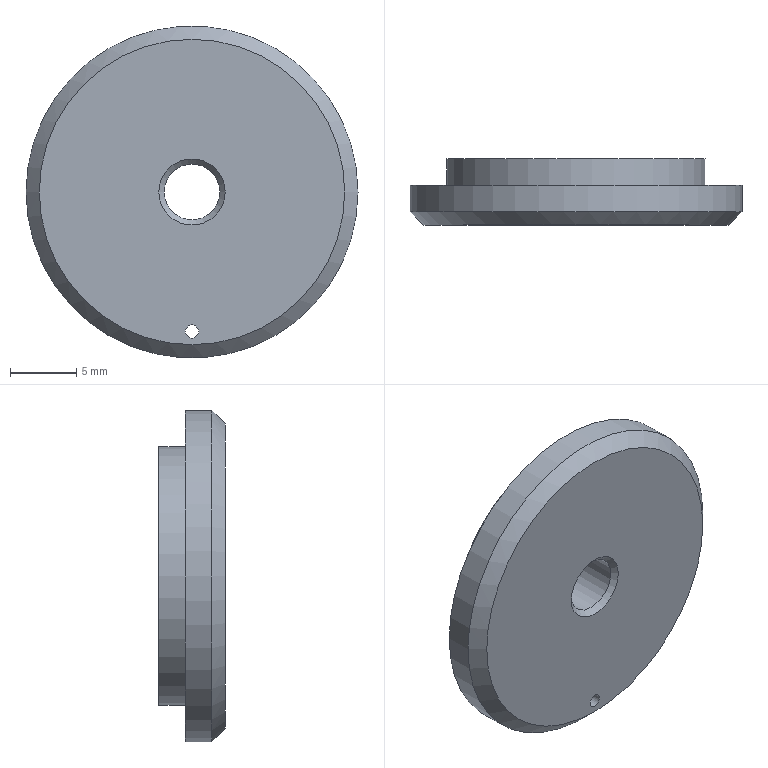Component | NX | 131_SHAFT_END_RING | 1 solid | 10 faces | box 25 x 5 x 25 mm | volume 1958 mm3 | cylinder 4 | plane 3 | cone 3 | commonest cylinder face diameters 19.5 x1 25 x1 1 x1 4.2 x1
STEP:
#1=CARTESIAN_POINT('',(0.,0.,0.));
#2=DIRECTION('',(0.,0.,1.));
#3=DIRECTION('',(1.,0.,0.));
#4=AXIS2_PLACEMENT_3D('',#1,#2,#3);
#5=CARTESIAN_POINT('',(-609.75,-183.7,-0.));
#6=VERTEX_POINT('',#5);
#7=CARTESIAN_POINT('',(-600.,-183.7,-0.));
#8=DIRECTION('',(0.,1.,0.));
#9=DIRECTION('',(-1.,0.,0.));
#10=AXIS2_PLACEMENT_3D('',#7,#8,#9);
#11=CIRCLE('',#10,9.75);
#12=CARTESIAN_POINT('',(-600.,-181.7,-0.));
#13=DIRECTION('',(0.,-1.,0.));
#14=DIRECTION('',(1.,0.,-0.));
#15=AXIS2_PLACEMENT_3D('',#12,#13,#14);
#16=CYLINDRICAL_SURFACE('',#15,9.75);
#17=CARTESIAN_POINT('',(9.425,2.));
#18=DIRECTION('',(-1.,0.));
#19=VECTOR('',#18,1.);
#20=LINE('',#17,#19);
#21=(GEOMETRIC_REPRESENTATION_CONTEXT(2)PARAMETRIC_REPRESENTATION_CONTEXT()REPRESENTATION_CONTEXT('',''));
#22=DEFINITIONAL_REPRESENTATION('',(#20),#21);
#23=PCURVE('',#16,#22);
#24=CARTESIAN_POINT('',(-600.,-183.7,-0.));
#25=DIRECTION('',(0.,1.,0.));
#26=DIRECTION('',(-1.,0.,0.));
#27=AXIS2_PLACEMENT_3D('',#24,#25,#26);
#28=PLANE('',#27);
#29=CARTESIAN_POINT('',(0.,0.));
#30=DIRECTION('',(1.,0.));
#31=AXIS2_PLACEMENT_2D('',#29,#30);
#32=CIRCLE('',#31,9.75);
#33=(GEOMETRIC_REPRESENTATION_CONTEXT(2)PARAMETRIC_REPRESENTATION_CONTEXT()REPRESENTATION_CONTEXT('',''));
#34=DEFINITIONAL_REPRESENTATION('',(#32),#33);
#35=PCURVE('',#28,#34);
#36=SURFACE_CURVE('',#11,(#23,#35),.PCURVE_S1.);
#37=EDGE_CURVE('',#6,#6,#36,.T.);
#38=ORIENTED_EDGE('',*,*,#37,.T.);
#39=CARTESIAN_POINT('',(-609.75,-181.7,-0.));
#40=VERTEX_POINT('',#39);
#41=CARTESIAN_POINT('',(-609.75,-181.7,-0.));
#42=CARTESIAN_POINT('',(-609.75,-183.7,-0.));
#43=B_SPLINE_CURVE_WITH_KNOTS('',1,(#41,#42),.UNSPECIFIED.,.F.,.F.,(2,2),(0.,2.),.PIECEWISE_BEZIER_KNOTS.);
#44=CARTESIAN_POINT('',(3.142,0.));
#45=DIRECTION('',(0.,1.));
#46=VECTOR('',#45,1.);
#47=LINE('',#44,#46);
#48=(GEOMETRIC_REPRESENTATION_CONTEXT(2)PARAMETRIC_REPRESENTATION_CONTEXT()REPRESENTATION_CONTEXT('',''));
#49=DEFINITIONAL_REPRESENTATION('',(#47),#48);
#50=PCURVE('',#16,#49);
#51=CARTESIAN_POINT('',(9.425,0.));
#52=DIRECTION('',(0.,1.));
#53=VECTOR('',#52,1.);
#54=LINE('',#51,#53);
#55=(GEOMETRIC_REPRESENTATION_CONTEXT(2)PARAMETRIC_REPRESENTATION_CONTEXT()REPRESENTATION_CONTEXT('',''));
#56=DEFINITIONAL_REPRESENTATION('',(#54),#55);
#57=PCURVE('',#16,#56);
#58=SEAM_CURVE('',#43,(#50,#57),.PCURVE_S1.);
#59=EDGE_CURVE('',#40,#6,#58,.T.);
#60=ORIENTED_EDGE('',*,*,#59,.F.);
#61=CARTESIAN_POINT('',(-600.,-181.7,-0.));
#62=DIRECTION('',(0.,1.,0.));
#63=DIRECTION('',(-1.,0.,0.));
#64=AXIS2_PLACEMENT_3D('',#61,#62,#63);
#65=CIRCLE('',#64,9.75);
#66=CARTESIAN_POINT('',(9.425,0.));
#67=DIRECTION('',(-1.,0.));
#68=VECTOR('',#67,1.);
#69=LINE('',#66,#68);
#70=(GEOMETRIC_REPRESENTATION_CONTEXT(2)PARAMETRIC_REPRESENTATION_CONTEXT()REPRESENTATION_CONTEXT('',''));
#71=DEFINITIONAL_REPRESENTATION('',(#69),#70);
#72=PCURVE('',#16,#71);
#73=CARTESIAN_POINT('',(-600.,-181.7,-0.));
#74=DIRECTION('',(0.,1.,0.));
#75=DIRECTION('',(-1.,0.,0.));
#76=AXIS2_PLACEMENT_3D('',#73,#74,#75);
#77=PLANE('',#76);
#78=CARTESIAN_POINT('',(0.,0.));
#79=DIRECTION('',(1.,0.));
#80=AXIS2_PLACEMENT_2D('',#78,#79);
#81=CIRCLE('',#80,9.75);
#82=(GEOMETRIC_REPRESENTATION_CONTEXT(2)PARAMETRIC_REPRESENTATION_CONTEXT()REPRESENTATION_CONTEXT('',''));
#83=DEFINITIONAL_REPRESENTATION('',(#81),#82);
#84=PCURVE('',#77,#83);
#85=SURFACE_CURVE('',#65,(#72,#84),.PCURVE_S1.);
#86=EDGE_CURVE('',#40,#40,#85,.T.);
#87=ORIENTED_EDGE('',*,*,#86,.F.);
#88=ORIENTED_EDGE('',*,*,#59,.T.);
#89=EDGE_LOOP('',(#38,#60,#87,#88));
#90=FACE_BOUND('',#89,.T.);
#91=ADVANCED_FACE('',(#90),#16,.T.);
#92=CARTESIAN_POINT('',(-602.5,-181.7,-0.));
#93=VERTEX_POINT('',#92);
#94=CARTESIAN_POINT('',(-600.,-181.7,-0.));
#95=DIRECTION('',(0.,-1.,0.));
#96=DIRECTION('',(-1.,0.,0.));
#97=AXIS2_PLACEMENT_3D('',#94,#95,#96);
#98=CIRCLE('',#97,2.5);
#99=CARTESIAN_POINT('',(2.5,0.));
#100=CARTESIAN_POINT('',(2.5,-4.33));
#101=CARTESIAN_POINT('',(-1.25,-2.165));
#102=CARTESIAN_POINT('',(-5.,-0.));
#103=CARTESIAN_POINT('',(-1.25,2.165));
#104=CARTESIAN_POINT('',(2.5,4.33));
#105=CARTESIAN_POINT('',(2.5,0.));
#106=(BOUNDED_CURVE()B_SPLINE_CURVE(2,(#99,#100,#101,#102,#103,#104,#105),.UNSPECIFIED.,.T.,.F.)B_SPLINE_CURVE_WITH_KNOTS((1,2,2,2,2,1),(-2.094,0.,2.094,4.189,6.283,8.378),.UNSPECIFIED.)CURVE()GEOMETRIC_REPRESENTATION_ITEM()RATIONAL_B_SPLINE_CURVE((1.,0.5,1.,0.5,1.,0.5,1.))REPRESENTATION_ITEM(''));
#107=(GEOMETRIC_REPRESENTATION_CONTEXT(2)PARAMETRIC_REPRESENTATION_CONTEXT()REPRESENTATION_CONTEXT('',''));
#108=DEFINITIONAL_REPRESENTATION('',(#106),#107);
#109=PCURVE('',#77,#108);
#110=CARTESIAN_POINT('',(-600.,-182.1,-0.));
#111=DIRECTION('',(0.,1.,0.));
#112=DIRECTION('',(-1.,0.,0.));
#113=AXIS2_PLACEMENT_3D('',#110,#111,#112);
#114=CONICAL_SURFACE('',#113,2.1,0.7854);
#115=CARTESIAN_POINT('',(6.283,0.4));
#116=DIRECTION('',(-1.,0.));
#117=VECTOR('',#116,1.);
#118=LINE('',#115,#117);
#119=(GEOMETRIC_REPRESENTATION_CONTEXT(2)PARAMETRIC_REPRESENTATION_CONTEXT()REPRESENTATION_CONTEXT('',''));
#120=DEFINITIONAL_REPRESENTATION('',(#118),#119);
#121=PCURVE('',#114,#120);
#122=SURFACE_CURVE('',#98,(#109,#121),.PCURVE_S1.);
#123=EDGE_CURVE('',#93,#93,#122,.T.);
#124=ORIENTED_EDGE('',*,*,#123,.T.);
#125=EDGE_LOOP('',(#124));
#126=FACE_BOUND('',#125,.T.);
#127=ORIENTED_EDGE('',*,*,#86,.T.);
#128=EDGE_LOOP('',(#127));
#129=FACE_BOUND('',#128,.T.);
#130=ADVANCED_FACE('',(#126,#129),#77,.T.);
#131=CARTESIAN_POINT('',(-612.5,-185.7,-0.));
#132=VERTEX_POINT('',#131);
#133=CARTESIAN_POINT('',(-600.,-185.7,-0.));
#134=DIRECTION('',(0.,1.,0.));
#135=DIRECTION('',(-1.,0.,0.));
#136=AXIS2_PLACEMENT_3D('',#133,#134,#135);
#137=CIRCLE('',#136,12.5);
#138=CARTESIAN_POINT('',(-600.,-183.7,-0.));
#139=DIRECTION('',(0.,-1.,0.));
#140=DIRECTION('',(1.,0.,-0.));
#141=AXIS2_PLACEMENT_3D('',#138,#139,#140);
#142=CYLINDRICAL_SURFACE('',#141,12.5);
#143=CARTESIAN_POINT('',(9.425,2.));
#144=DIRECTION('',(-1.,0.));
#145=VECTOR('',#144,1.);
#146=LINE('',#143,#145);
#147=(GEOMETRIC_REPRESENTATION_CONTEXT(2)PARAMETRIC_REPRESENTATION_CONTEXT()REPRESENTATION_CONTEXT('',''));
#148=DEFINITIONAL_REPRESENTATION('',(#146),#147);
#149=PCURVE('',#142,#148);
#150=CARTESIAN_POINT('',(-600.,-185.7,-0.));
#151=DIRECTION('',(0.,1.,0.));
#152=DIRECTION('',(-1.,0.,0.));
#153=AXIS2_PLACEMENT_3D('',#150,#151,#152);
#154=CONICAL_SURFACE('',#153,12.5,0.7854);
#155=CARTESIAN_POINT('',(0.,0.));
#156=DIRECTION('',(1.,0.));
#157=VECTOR('',#156,1.);
#158=LINE('',#155,#157);
#159=(GEOMETRIC_REPRESENTATION_CONTEXT(2)PARAMETRIC_REPRESENTATION_CONTEXT()REPRESENTATION_CONTEXT('',''));
#160=DEFINITIONAL_REPRESENTATION('',(#158),#159);
#161=PCURVE('',#154,#160);
#162=SURFACE_CURVE('',#137,(#149,#161),.PCURVE_S1.);
#163=EDGE_CURVE('',#132,#132,#162,.T.);
#164=ORIENTED_EDGE('',*,*,#163,.T.);
#165=CARTESIAN_POINT('',(-612.5,-183.7,-0.));
#166=VERTEX_POINT('',#165);
#167=CARTESIAN_POINT('',(-612.5,-183.7,-0.));
#168=CARTESIAN_POINT('',(-612.5,-185.7,-0.));
#169=B_SPLINE_CURVE_WITH_KNOTS('',1,(#167,#168),.UNSPECIFIED.,.F.,.F.,(2,2),(0.,2.),.PIECEWISE_BEZIER_KNOTS.);
#170=CARTESIAN_POINT('',(3.142,0.));
#171=DIRECTION('',(0.,1.));
#172=VECTOR('',#171,1.);
#173=LINE('',#170,#172);
#174=(GEOMETRIC_REPRESENTATION_CONTEXT(2)PARAMETRIC_REPRESENTATION_CONTEXT()REPRESENTATION_CONTEXT('',''));
#175=DEFINITIONAL_REPRESENTATION('',(#173),#174);
#176=PCURVE('',#142,#175);
#177=CARTESIAN_POINT('',(9.425,0.));
#178=DIRECTION('',(0.,1.));
#179=VECTOR('',#178,1.);
#180=LINE('',#177,#179);
#181=(GEOMETRIC_REPRESENTATION_CONTEXT(2)PARAMETRIC_REPRESENTATION_CONTEXT()REPRESENTATION_CONTEXT('',''));
#182=DEFINITIONAL_REPRESENTATION('',(#180),#181);
#183=PCURVE('',#142,#182);
#184=SEAM_CURVE('',#169,(#176,#183),.PCURVE_S1.);
#185=EDGE_CURVE('',#166,#132,#184,.T.);
#186=ORIENTED_EDGE('',*,*,#185,.F.);
#187=CARTESIAN_POINT('',(-600.,-183.7,-0.));
#188=DIRECTION('',(0.,1.,0.));
#189=DIRECTION('',(-1.,0.,0.));
#190=AXIS2_PLACEMENT_3D('',#187,#188,#189);
#191=CIRCLE('',#190,12.5);
#192=CARTESIAN_POINT('',(9.425,0.));
#193=DIRECTION('',(-1.,0.));
#194=VECTOR('',#193,1.);
#195=LINE('',#192,#194);
#196=(GEOMETRIC_REPRESENTATION_CONTEXT(2)PARAMETRIC_REPRESENTATION_CONTEXT()REPRESENTATION_CONTEXT('',''));
#197=DEFINITIONAL_REPRESENTATION('',(#195),#196);
#198=PCURVE('',#142,#197);
#199=CARTESIAN_POINT('',(0.,0.));
#200=DIRECTION('',(1.,0.));
#201=AXIS2_PLACEMENT_2D('',#199,#200);
#202=CIRCLE('',#201,12.5);
#203=(GEOMETRIC_REPRESENTATION_CONTEXT(2)PARAMETRIC_REPRESENTATION_CONTEXT()REPRESENTATION_CONTEXT('',''));
#204=DEFINITIONAL_REPRESENTATION('',(#202),#203);
#205=PCURVE('',#28,#204);
#206=SURFACE_CURVE('',#191,(#198,#205),.PCURVE_S1.);
#207=EDGE_CURVE('',#166,#166,#206,.T.);
#208=ORIENTED_EDGE('',*,*,#207,.F.);
#209=ORIENTED_EDGE('',*,*,#185,.T.);
#210=EDGE_LOOP('',(#164,#186,#208,#209));
#211=FACE_BOUND('',#210,.T.);
#212=ADVANCED_FACE('',(#211),#142,.T.);
#213=CARTESIAN_POINT('',(-600.5,-183.7,-10.5));
#214=VERTEX_POINT('',#213);
#215=CARTESIAN_POINT('',(-600.,-183.7,-10.5));
#216=DIRECTION('',(0.,1.,0.));
#217=DIRECTION('',(-1.,0.,0.));
#218=AXIS2_PLACEMENT_3D('',#215,#216,#217);
#219=CIRCLE('',#218,0.5);
#220=CARTESIAN_POINT('',(0.,-10.5));
#221=DIRECTION('',(1.,0.));
#222=AXIS2_PLACEMENT_2D('',#220,#221);
#223=CIRCLE('',#222,0.5);
#224=(GEOMETRIC_REPRESENTATION_CONTEXT(2)PARAMETRIC_REPRESENTATION_CONTEXT()REPRESENTATION_CONTEXT('',''));
#225=DEFINITIONAL_REPRESENTATION('',(#223),#224);
#226=PCURVE('',#28,#225);
#227=CARTESIAN_POINT('',(-600.,-181.7,-10.5));
#228=DIRECTION('',(0.,-1.,0.));
#229=DIRECTION('',(1.,0.,-0.));
#230=AXIS2_PLACEMENT_3D('',#227,#228,#229);
#231=CYLINDRICAL_SURFACE('',#230,0.5);
#232=CARTESIAN_POINT('',(9.425,2.));
#233=DIRECTION('',(-1.,0.));
#234=VECTOR('',#233,1.);
#235=LINE('',#232,#234);
#236=(GEOMETRIC_REPRESENTATION_CONTEXT(2)PARAMETRIC_REPRESENTATION_CONTEXT()REPRESENTATION_CONTEXT('',''));
#237=DEFINITIONAL_REPRESENTATION('',(#235),#236);
#238=PCURVE('',#231,#237);
#239=SURFACE_CURVE('',#219,(#226,#238),.PCURVE_S1.);
#240=EDGE_CURVE('',#214,#214,#239,.T.);
#241=ORIENTED_EDGE('',*,*,#240,.F.);
#242=EDGE_LOOP('',(#241));
#243=FACE_BOUND('',#242,.T.);
#244=ORIENTED_EDGE('',*,*,#207,.T.);
#245=EDGE_LOOP('',(#244));
#246=FACE_BOUND('',#245,.T.);
#247=ORIENTED_EDGE('',*,*,#37,.F.);
#248=EDGE_LOOP('',(#247));
#249=FACE_BOUND('',#248,.T.);
#250=ADVANCED_FACE('',(#243,#246,#249),#28,.T.);
#251=CARTESIAN_POINT('',(-602.5,-186.7,-0.));
#252=VERTEX_POINT('',#251);
#253=CARTESIAN_POINT('',(-600.,-186.7,-0.));
#254=DIRECTION('',(0.,1.,0.));
#255=DIRECTION('',(-1.,0.,0.));
#256=AXIS2_PLACEMENT_3D('',#253,#254,#255);
#257=CIRCLE('',#256,2.5);
#258=CARTESIAN_POINT('',(-600.,-186.7,-0.));
#259=DIRECTION('',(0.,1.,0.));
#260=DIRECTION('',(-1.,0.,0.));
#261=AXIS2_PLACEMENT_3D('',#258,#259,#260);
#262=PLANE('',#261);
#263=CARTESIAN_POINT('',(0.,0.));
#264=DIRECTION('',(1.,0.));
#265=AXIS2_PLACEMENT_2D('',#263,#264);
#266=CIRCLE('',#265,2.5);
#267=(GEOMETRIC_REPRESENTATION_CONTEXT(2)PARAMETRIC_REPRESENTATION_CONTEXT()REPRESENTATION_CONTEXT('',''));
#268=DEFINITIONAL_REPRESENTATION('',(#266),#267);
#269=PCURVE('',#262,#268);
#270=CARTESIAN_POINT('',(-600.,-186.7,-0.));
#271=DIRECTION('',(0.,-1.,0.));
#272=DIRECTION('',(1.,0.,-0.));
#273=AXIS2_PLACEMENT_3D('',#270,#271,#272);
#274=CONICAL_SURFACE('',#273,2.5,0.7854);
#275=CARTESIAN_POINT('',(9.425,0.));
#276=DIRECTION('',(-1.,0.));
#277=VECTOR('',#276,1.);
#278=LINE('',#275,#277);
#279=(GEOMETRIC_REPRESENTATION_CONTEXT(2)PARAMETRIC_REPRESENTATION_CONTEXT()REPRESENTATION_CONTEXT('',''));
#280=DEFINITIONAL_REPRESENTATION('',(#278),#279);
#281=PCURVE('',#274,#280);
#282=SURFACE_CURVE('',#257,(#269,#281),.PCURVE_S1.);
#283=EDGE_CURVE('',#252,#252,#282,.T.);
#284=ORIENTED_EDGE('',*,*,#283,.T.);
#285=EDGE_LOOP('',(#284));
#286=FACE_BOUND('',#285,.T.);
#287=CARTESIAN_POINT('',(-600.5,-186.7,-10.5));
#288=VERTEX_POINT('',#287);
#289=CARTESIAN_POINT('',(-600.,-186.7,-10.5));
#290=DIRECTION('',(0.,-1.,0.));
#291=DIRECTION('',(-1.,0.,0.));
#292=AXIS2_PLACEMENT_3D('',#289,#290,#291);
#293=CIRCLE('',#292,0.5);
#294=CARTESIAN_POINT('',(0.5,-10.5));
#295=CARTESIAN_POINT('',(0.5,-11.366));
#296=CARTESIAN_POINT('',(-0.25,-10.933));
#297=CARTESIAN_POINT('',(-1.,-10.5));
#298=CARTESIAN_POINT('',(-0.25,-10.067));
#299=CARTESIAN_POINT('',(0.5,-9.634));
#300=CARTESIAN_POINT('',(0.5,-10.5));
#301=(BOUNDED_CURVE()B_SPLINE_CURVE(2,(#294,#295,#296,#297,#298,#299,#300),.UNSPECIFIED.,.T.,.F.)B_SPLINE_CURVE_WITH_KNOTS((1,2,2,2,2,1),(-2.094,0.,2.094,4.189,6.283,8.378),.UNSPECIFIED.)CURVE()GEOMETRIC_REPRESENTATION_ITEM()RATIONAL_B_SPLINE_CURVE((1.,0.5,1.,0.5,1.,0.5,1.))REPRESENTATION_ITEM(''));
#302=(GEOMETRIC_REPRESENTATION_CONTEXT(2)PARAMETRIC_REPRESENTATION_CONTEXT()REPRESENTATION_CONTEXT('',''));
#303=DEFINITIONAL_REPRESENTATION('',(#301),#302);
#304=PCURVE('',#262,#303);
#305=CARTESIAN_POINT('',(3.142,5.));
#306=DIRECTION('',(1.,0.));
#307=VECTOR('',#306,1.);
#308=LINE('',#305,#307);
#309=(GEOMETRIC_REPRESENTATION_CONTEXT(2)PARAMETRIC_REPRESENTATION_CONTEXT()REPRESENTATION_CONTEXT('',''));
#310=DEFINITIONAL_REPRESENTATION('',(#308),#309);
#311=PCURVE('',#231,#310);
#312=SURFACE_CURVE('',#293,(#304,#311),.PCURVE_S1.);
#313=EDGE_CURVE('',#288,#288,#312,.T.);
#314=ORIENTED_EDGE('',*,*,#313,.F.);
#315=EDGE_LOOP('',(#314));
#316=FACE_BOUND('',#315,.T.);
#317=CARTESIAN_POINT('',(-611.5,-186.7,-0.));
#318=VERTEX_POINT('',#317);
#319=CARTESIAN_POINT('',(-600.,-186.7,-0.));
#320=DIRECTION('',(0.,-1.,0.));
#321=DIRECTION('',(-1.,0.,0.));
#322=AXIS2_PLACEMENT_3D('',#319,#320,#321);
#323=CIRCLE('',#322,11.5);
#324=CARTESIAN_POINT('',(11.5,0.));
#325=CARTESIAN_POINT('',(11.5,-19.919));
#326=CARTESIAN_POINT('',(-5.75,-9.959));
#327=CARTESIAN_POINT('',(-23.,-0.));
#328=CARTESIAN_POINT('',(-5.75,9.959));
#329=CARTESIAN_POINT('',(11.5,19.919));
#330=CARTESIAN_POINT('',(11.5,0.));
#331=(BOUNDED_CURVE()B_SPLINE_CURVE(2,(#324,#325,#326,#327,#328,#329,#330),.UNSPECIFIED.,.T.,.F.)B_SPLINE_CURVE_WITH_KNOTS((1,2,2,2,2,1),(-2.094,0.,2.094,4.189,6.283,8.378),.UNSPECIFIED.)CURVE()GEOMETRIC_REPRESENTATION_ITEM()RATIONAL_B_SPLINE_CURVE((1.,0.5,1.,0.5,1.,0.5,1.))REPRESENTATION_ITEM(''));
#332=(GEOMETRIC_REPRESENTATION_CONTEXT(2)PARAMETRIC_REPRESENTATION_CONTEXT()REPRESENTATION_CONTEXT('',''));
#333=DEFINITIONAL_REPRESENTATION('',(#331),#332);
#334=PCURVE('',#262,#333);
#335=CARTESIAN_POINT('',(6.283,-1.));
#336=DIRECTION('',(-1.,0.));
#337=VECTOR('',#336,1.);
#338=LINE('',#335,#337);
#339=(GEOMETRIC_REPRESENTATION_CONTEXT(2)PARAMETRIC_REPRESENTATION_CONTEXT()REPRESENTATION_CONTEXT('',''));
#340=DEFINITIONAL_REPRESENTATION('',(#338),#339);
#341=PCURVE('',#154,#340);
#342=SURFACE_CURVE('',#323,(#334,#341),.PCURVE_S1.);
#343=EDGE_CURVE('',#318,#318,#342,.T.);
#344=ORIENTED_EDGE('',*,*,#343,.T.);
#345=EDGE_LOOP('',(#344));
#346=FACE_BOUND('',#345,.T.);
#347=ADVANCED_FACE('',(#286,#316,#346),#262,.F.);
#348=ORIENTED_EDGE('',*,*,#343,.F.);
#349=CARTESIAN_POINT('',(-611.5,-186.7,-0.));
#350=CARTESIAN_POINT('',(-612.5,-185.7,-0.));
#351=B_SPLINE_CURVE_WITH_KNOTS('',1,(#349,#350),.UNSPECIFIED.,.F.,.F.,(2,2),(-1.414,0.),.PIECEWISE_BEZIER_KNOTS.);
#352=CARTESIAN_POINT('',(6.283,0.));
#353=DIRECTION('',(0.,1.));
#354=VECTOR('',#353,1.);
#355=LINE('',#352,#354);
#356=(GEOMETRIC_REPRESENTATION_CONTEXT(2)PARAMETRIC_REPRESENTATION_CONTEXT()REPRESENTATION_CONTEXT('',''));
#357=DEFINITIONAL_REPRESENTATION('',(#355),#356);
#358=PCURVE('',#154,#357);
#359=CARTESIAN_POINT('',(0.,0.));
#360=DIRECTION('',(0.,1.));
#361=VECTOR('',#360,1.);
#362=LINE('',#359,#361);
#363=(GEOMETRIC_REPRESENTATION_CONTEXT(2)PARAMETRIC_REPRESENTATION_CONTEXT()REPRESENTATION_CONTEXT('',''));
#364=DEFINITIONAL_REPRESENTATION('',(#362),#363);
#365=PCURVE('',#154,#364);
#366=SEAM_CURVE('',#351,(#358,#365),.PCURVE_S1.);
#367=EDGE_CURVE('',#318,#132,#366,.T.);
#368=ORIENTED_EDGE('',*,*,#367,.T.);
#369=ORIENTED_EDGE('',*,*,#163,.F.);
#370=ORIENTED_EDGE('',*,*,#367,.F.);
#371=EDGE_LOOP('',(#348,#368,#369,#370));
#372=FACE_BOUND('',#371,.T.);
#373=ADVANCED_FACE('',(#372),#154,.T.);
#374=ORIENTED_EDGE('',*,*,#240,.F.);
#375=CARTESIAN_POINT('',(-600.5,-183.7,-10.5));
#376=CARTESIAN_POINT('',(-600.5,-186.7,-10.5));
#377=B_SPLINE_CURVE_WITH_KNOTS('',1,(#375,#376),.UNSPECIFIED.,.F.,.F.,(2,2),(2.,5.),.PIECEWISE_BEZIER_KNOTS.);
#378=CARTESIAN_POINT('',(9.425,0.));
#379=DIRECTION('',(0.,1.));
#380=VECTOR('',#379,1.);
#381=LINE('',#378,#380);
#382=(GEOMETRIC_REPRESENTATION_CONTEXT(2)PARAMETRIC_REPRESENTATION_CONTEXT()REPRESENTATION_CONTEXT('',''));
#383=DEFINITIONAL_REPRESENTATION('',(#381),#382);
#384=PCURVE('',#231,#383);
#385=CARTESIAN_POINT('',(3.142,0.));
#386=DIRECTION('',(0.,1.));
#387=VECTOR('',#386,1.);
#388=LINE('',#385,#387);
#389=(GEOMETRIC_REPRESENTATION_CONTEXT(2)PARAMETRIC_REPRESENTATION_CONTEXT()REPRESENTATION_CONTEXT('',''));
#390=DEFINITIONAL_REPRESENTATION('',(#388),#389);
#391=PCURVE('',#231,#390);
#392=SEAM_CURVE('',#377,(#384,#391),.PCURVE_S1.);
#393=EDGE_CURVE('',#214,#288,#392,.T.);
#394=ORIENTED_EDGE('',*,*,#393,.T.);
#395=ORIENTED_EDGE('',*,*,#313,.F.);
#396=ORIENTED_EDGE('',*,*,#393,.F.);
#397=EDGE_LOOP('',(#374,#394,#395,#396));
#398=FACE_BOUND('',#397,.F.);
#399=ADVANCED_FACE('',(#398),#231,.F.);
#400=CARTESIAN_POINT('',(-602.1,-182.1,-0.));
#401=VERTEX_POINT('',#400);
#402=CARTESIAN_POINT('',(-600.,-182.1,-0.));
#403=DIRECTION('',(0.,1.,0.));
#404=DIRECTION('',(-1.,0.,0.));
#405=AXIS2_PLACEMENT_3D('',#402,#403,#404);
#406=CIRCLE('',#405,2.1);
#407=CARTESIAN_POINT('',(-600.,-186.7,-0.));
#408=DIRECTION('',(0.,1.,0.));
#409=DIRECTION('',(-1.,0.,0.));
#410=AXIS2_PLACEMENT_3D('',#407,#408,#409);
#411=CYLINDRICAL_SURFACE('',#410,2.1);
#412=CARTESIAN_POINT('',(0.,4.6));
#413=DIRECTION('',(1.,0.));
#414=VECTOR('',#413,1.);
#415=LINE('',#412,#414);
#416=(GEOMETRIC_REPRESENTATION_CONTEXT(2)PARAMETRIC_REPRESENTATION_CONTEXT()REPRESENTATION_CONTEXT('',''));
#417=DEFINITIONAL_REPRESENTATION('',(#415),#416);
#418=PCURVE('',#411,#417);
#419=CARTESIAN_POINT('',(0.,0.));
#420=DIRECTION('',(1.,0.));
#421=VECTOR('',#420,1.);
#422=LINE('',#419,#421);
#423=(GEOMETRIC_REPRESENTATION_CONTEXT(2)PARAMETRIC_REPRESENTATION_CONTEXT()REPRESENTATION_CONTEXT('',''));
#424=DEFINITIONAL_REPRESENTATION('',(#422),#423);
#425=PCURVE('',#114,#424);
#426=SURFACE_CURVE('',#406,(#418,#425),.PCURVE_S1.);
#427=EDGE_CURVE('',#401,#401,#426,.T.);
#428=ORIENTED_EDGE('',*,*,#427,.F.);
#429=CARTESIAN_POINT('',(-602.1,-186.3,-0.));
#430=VERTEX_POINT('',#429);
#431=CARTESIAN_POINT('',(-602.1,-186.3,-0.));
#432=CARTESIAN_POINT('',(-602.1,-182.1,-0.));
#433=B_SPLINE_CURVE_WITH_KNOTS('',1,(#431,#432),.UNSPECIFIED.,.F.,.F.,(2,2),(0.4,4.6),.PIECEWISE_BEZIER_KNOTS.);
#434=CARTESIAN_POINT('',(0.,0.));
#435=DIRECTION('',(0.,1.));
#436=VECTOR('',#435,1.);
#437=LINE('',#434,#436);
#438=(GEOMETRIC_REPRESENTATION_CONTEXT(2)PARAMETRIC_REPRESENTATION_CONTEXT()REPRESENTATION_CONTEXT('',''));
#439=DEFINITIONAL_REPRESENTATION('',(#437),#438);
#440=PCURVE('',#411,#439);
#441=CARTESIAN_POINT('',(6.283,0.));
#442=DIRECTION('',(0.,1.));
#443=VECTOR('',#442,1.);
#444=LINE('',#441,#443);
#445=(GEOMETRIC_REPRESENTATION_CONTEXT(2)PARAMETRIC_REPRESENTATION_CONTEXT()REPRESENTATION_CONTEXT('',''));
#446=DEFINITIONAL_REPRESENTATION('',(#444),#445);
#447=PCURVE('',#411,#446);
#448=SEAM_CURVE('',#433,(#440,#447),.PCURVE_S1.);
#449=EDGE_CURVE('',#430,#401,#448,.T.);
#450=ORIENTED_EDGE('',*,*,#449,.F.);
#451=CARTESIAN_POINT('',(-600.,-186.3,-0.));
#452=DIRECTION('',(0.,-1.,0.));
#453=DIRECTION('',(-1.,0.,0.));
#454=AXIS2_PLACEMENT_3D('',#451,#452,#453);
#455=CIRCLE('',#454,2.1);
#456=CARTESIAN_POINT('',(6.283,0.4));
#457=DIRECTION('',(-1.,0.));
#458=VECTOR('',#457,1.);
#459=LINE('',#456,#458);
#460=(GEOMETRIC_REPRESENTATION_CONTEXT(2)PARAMETRIC_REPRESENTATION_CONTEXT()REPRESENTATION_CONTEXT('',''));
#461=DEFINITIONAL_REPRESENTATION('',(#459),#460);
#462=PCURVE('',#411,#461);
#463=CARTESIAN_POINT('',(3.142,-0.4));
#464=DIRECTION('',(1.,0.));
#465=VECTOR('',#464,1.);
#466=LINE('',#463,#465);
#467=(GEOMETRIC_REPRESENTATION_CONTEXT(2)PARAMETRIC_REPRESENTATION_CONTEXT()REPRESENTATION_CONTEXT('',''));
#468=DEFINITIONAL_REPRESENTATION('',(#466),#467);
#469=PCURVE('',#274,#468);
#470=SURFACE_CURVE('',#455,(#462,#469),.PCURVE_S1.);
#471=EDGE_CURVE('',#430,#430,#470,.T.);
#472=ORIENTED_EDGE('',*,*,#471,.F.);
#473=ORIENTED_EDGE('',*,*,#449,.T.);
#474=EDGE_LOOP('',(#428,#450,#472,#473));
#475=FACE_BOUND('',#474,.F.);
#476=ADVANCED_FACE('',(#475),#411,.F.);
#477=ORIENTED_EDGE('',*,*,#471,.T.);
#478=CARTESIAN_POINT('',(-602.1,-186.3,-0.));
#479=CARTESIAN_POINT('',(-602.5,-186.7,-0.));
#480=B_SPLINE_CURVE_WITH_KNOTS('',1,(#478,#479),.UNSPECIFIED.,.F.,.F.,(2,2),(-0.5657,0.),.PIECEWISE_BEZIER_KNOTS.);
#481=CARTESIAN_POINT('',(9.425,0.));
#482=DIRECTION('',(0.,1.));
#483=VECTOR('',#482,1.);
#484=LINE('',#481,#483);
#485=(GEOMETRIC_REPRESENTATION_CONTEXT(2)PARAMETRIC_REPRESENTATION_CONTEXT()REPRESENTATION_CONTEXT('',''));
#486=DEFINITIONAL_REPRESENTATION('',(#484),#485);
#487=PCURVE('',#274,#486);
#488=CARTESIAN_POINT('',(3.142,0.));
#489=DIRECTION('',(0.,1.));
#490=VECTOR('',#489,1.);
#491=LINE('',#488,#490);
#492=(GEOMETRIC_REPRESENTATION_CONTEXT(2)PARAMETRIC_REPRESENTATION_CONTEXT()REPRESENTATION_CONTEXT('',''));
#493=DEFINITIONAL_REPRESENTATION('',(#491),#492);
#494=PCURVE('',#274,#493);
#495=SEAM_CURVE('',#480,(#487,#494),.PCURVE_S1.);
#496=EDGE_CURVE('',#430,#252,#495,.T.);
#497=ORIENTED_EDGE('',*,*,#496,.T.);
#498=ORIENTED_EDGE('',*,*,#283,.T.);
#499=ORIENTED_EDGE('',*,*,#496,.F.);
#500=EDGE_LOOP('',(#477,#497,#498,#499));
#501=FACE_BOUND('',#500,.F.);
#502=ADVANCED_FACE('',(#501),#274,.F.);
#503=ORIENTED_EDGE('',*,*,#123,.T.);
#504=CARTESIAN_POINT('',(-602.1,-182.1,-0.));
#505=CARTESIAN_POINT('',(-602.5,-181.7,-0.));
#506=B_SPLINE_CURVE_WITH_KNOTS('',1,(#504,#505),.UNSPECIFIED.,.F.,.F.,(2,2),(0.,0.5657),.PIECEWISE_BEZIER_KNOTS.);
#507=CARTESIAN_POINT('',(0.,0.));
#508=DIRECTION('',(0.,1.));
#509=VECTOR('',#508,1.);
#510=LINE('',#507,#509);
#511=(GEOMETRIC_REPRESENTATION_CONTEXT(2)PARAMETRIC_REPRESENTATION_CONTEXT()REPRESENTATION_CONTEXT('',''));
#512=DEFINITIONAL_REPRESENTATION('',(#510),#511);
#513=PCURVE('',#114,#512);
#514=CARTESIAN_POINT('',(6.283,0.));
#515=DIRECTION('',(0.,1.));
#516=VECTOR('',#515,1.);
#517=LINE('',#514,#516);
#518=(GEOMETRIC_REPRESENTATION_CONTEXT(2)PARAMETRIC_REPRESENTATION_CONTEXT()REPRESENTATION_CONTEXT('',''));
#519=DEFINITIONAL_REPRESENTATION('',(#517),#518);
#520=PCURVE('',#114,#519);
#521=SEAM_CURVE('',#506,(#513,#520),.PCURVE_S1.);
#522=EDGE_CURVE('',#401,#93,#521,.T.);
#523=ORIENTED_EDGE('',*,*,#522,.F.);
#524=ORIENTED_EDGE('',*,*,#427,.T.);
#525=ORIENTED_EDGE('',*,*,#522,.T.);
#526=EDGE_LOOP('',(#503,#523,#524,#525));
#527=FACE_BOUND('',#526,.F.);
#528=ADVANCED_FACE('',(#527),#114,.F.);
#529=CLOSED_SHELL('',(#91,#130,#212,#250,#347,#373,#399,#476,#502,#528));
#530=MANIFOLD_SOLID_BREP('',#529);
#531=(LENGTH_UNIT()NAMED_UNIT(*)SI_UNIT(.MILLI.,.METRE.));
#532=UNCERTAINTY_MEASURE_WITH_UNIT(LENGTH_MEASURE(0.00001),#531,'','');
#533=(NAMED_UNIT(*)PLANE_ANGLE_UNIT()SI_UNIT($,.RADIAN.));
#534=(NAMED_UNIT(*)SI_UNIT($,.STERADIAN.)SOLID_ANGLE_UNIT());
#535=(GEOMETRIC_REPRESENTATION_CONTEXT(3)GLOBAL_UNCERTAINTY_ASSIGNED_CONTEXT((#532))GLOBAL_UNIT_ASSIGNED_CONTEXT((#531,#533,#534))REPRESENTATION_CONTEXT('',''));
#536=ADVANCED_BREP_SHAPE_REPRESENTATION('',(#4,#530),#535);